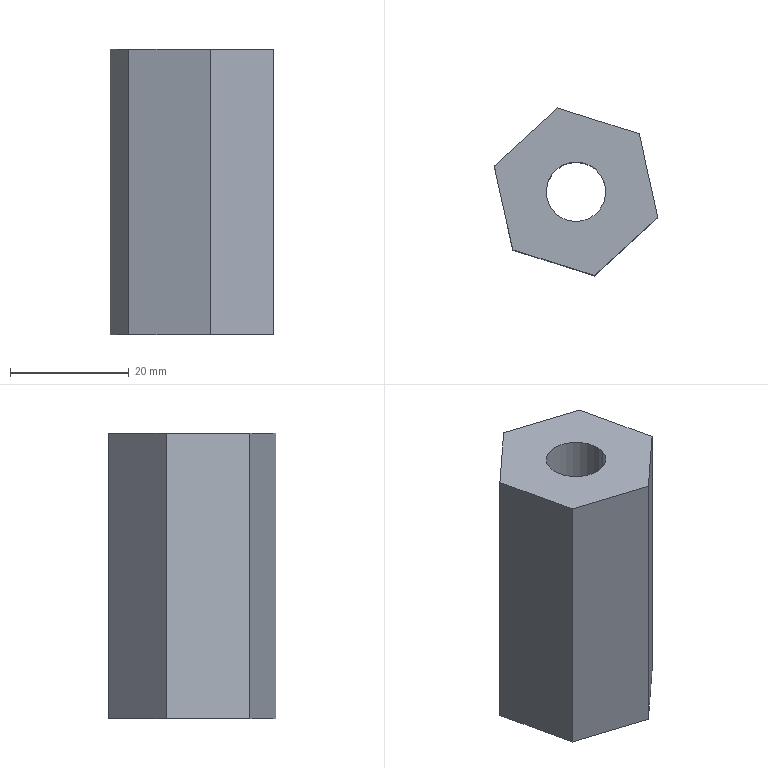Component | SolidWorks | ScraperSupport-1 | 1 solid | 10 faces | box 27.53 x 28.18 x 48 mm | volume 22211 mm3 | plane 8 | cylinder 2 | commonest cylinder face diameters 10 x2
STEP:
#1=COLOUR_RGB('',0.7922,0.8196,0.9333);
#2=FILL_AREA_STYLE_COLOUR('',#1);
#3=FILL_AREA_STYLE('',(#2));
#4=SURFACE_STYLE_FILL_AREA(#3);
#5=SURFACE_SIDE_STYLE('',(#4));
#6=SURFACE_STYLE_USAGE(.BOTH.,#5);
#7=PRESENTATION_STYLE_ASSIGNMENT((#6));
#8=CARTESIAN_POINT('',(20.038,-9.226,57.903));
#9=VERTEX_POINT('',#8);
#10=CARTESIAN_POINT('',(19.666,-9.098,57.903));
#11=VERTEX_POINT('',#10);
#12=CARTESIAN_POINT('',(19.852,-9.162,57.903));
#13=DIRECTION('',(-0.,-0.,-1.));
#14=DIRECTION('',(-0.9451,0.3269,0.));
#15=AXIS2_PLACEMENT_3D('',#12,#13,#14);
#16=CIRCLE('',#15,0.1969);
#17=EDGE_CURVE('',#9,#11,#16,.T.);
#18=ORIENTED_EDGE('',*,*,#17,.T.);
#19=CARTESIAN_POINT('',(19.666,-9.098,59.792));
#20=VERTEX_POINT('',#19);
#21=CARTESIAN_POINT('',(19.666,-9.098,57.903));
#22=DIRECTION('',(0.,0.,1.));
#23=VECTOR('',#22,39.37);
#24=LINE('',#21,#23);
#25=EDGE_CURVE('',#11,#20,#24,.T.);
#26=ORIENTED_EDGE('',*,*,#25,.T.);
#27=CARTESIAN_POINT('',(20.038,-9.226,59.792));
#28=VERTEX_POINT('',#27);
#29=CARTESIAN_POINT('',(19.852,-9.162,59.792));
#30=DIRECTION('',(-0.,-0.,-1.));
#31=DIRECTION('',(-0.9451,0.3269,0.));
#32=AXIS2_PLACEMENT_3D('',#29,#30,#31);
#33=CIRCLE('',#32,0.1969);
#34=EDGE_CURVE('',#28,#20,#33,.T.);
#35=ORIENTED_EDGE('',*,*,#34,.F.);
#36=CARTESIAN_POINT('',(20.038,-9.226,57.903));
#37=DIRECTION('',(0.,0.,1.));
#38=VECTOR('',#37,39.37);
#39=LINE('',#36,#38);
#40=EDGE_CURVE('',#9,#28,#39,.T.);
#41=ORIENTED_EDGE('',*,*,#40,.F.);
#42=EDGE_LOOP('',(#18,#26,#35,#41));
#43=FACE_OUTER_BOUND('',#42,.T.);
#44=CARTESIAN_POINT('',(19.852,-9.162,57.903));
#45=DIRECTION('',(0.,0.,1.));
#46=DIRECTION('',(0.9451,-0.3269,0.));
#47=AXIS2_PLACEMENT_3D('',#44,#45,#46);
#48=CYLINDRICAL_SURFACE('',#47,0.1969);
#49=ADVANCED_FACE('',(#43),#48,.F.);
#50=CARTESIAN_POINT('',(19.31,-8.991,57.903));
#51=VERTEX_POINT('',#50);
#52=CARTESIAN_POINT('',(19.729,-8.607,57.903));
#53=VERTEX_POINT('',#52);
#54=CARTESIAN_POINT('',(19.31,-8.991,57.903));
#55=DIRECTION('',(0.7374,0.6754,-0.));
#56=VECTOR('',#55,39.37);
#57=LINE('',#54,#56);
#58=EDGE_CURVE('',#51,#53,#57,.T.);
#59=ORIENTED_EDGE('',*,*,#58,.T.);
#60=CARTESIAN_POINT('',(20.271,-8.778,57.903));
#61=VERTEX_POINT('',#60);
#62=CARTESIAN_POINT('',(19.729,-8.607,57.903));
#63=DIRECTION('',(0.9537,-0.3009,-0.));
#64=VECTOR('',#63,39.37);
#65=LINE('',#62,#64);
#66=EDGE_CURVE('',#53,#61,#65,.T.);
#67=ORIENTED_EDGE('',*,*,#66,.T.);
#68=CARTESIAN_POINT('',(20.394,-9.333,57.903));
#69=VERTEX_POINT('',#68);
#70=CARTESIAN_POINT('',(20.271,-8.778,57.903));
#71=DIRECTION('',(0.2162,-0.9763,0.));
#72=VECTOR('',#71,39.37);
#73=LINE('',#70,#72);
#74=EDGE_CURVE('',#61,#69,#73,.T.);
#75=ORIENTED_EDGE('',*,*,#74,.T.);
#76=CARTESIAN_POINT('',(19.975,-9.717,57.903));
#77=VERTEX_POINT('',#76);
#78=CARTESIAN_POINT('',(20.394,-9.333,57.903));
#79=DIRECTION('',(-0.7374,-0.6754,0.));
#80=VECTOR('',#79,39.37);
#81=LINE('',#78,#80);
#82=EDGE_CURVE('',#69,#77,#81,.T.);
#83=ORIENTED_EDGE('',*,*,#82,.T.);
#84=CARTESIAN_POINT('',(19.433,-9.546,57.903));
#85=VERTEX_POINT('',#84);
#86=CARTESIAN_POINT('',(19.975,-9.717,57.903));
#87=DIRECTION('',(-0.9537,0.3009,0.));
#88=VECTOR('',#87,39.37);
#89=LINE('',#86,#88);
#90=EDGE_CURVE('',#77,#85,#89,.T.);
#91=ORIENTED_EDGE('',*,*,#90,.T.);
#92=CARTESIAN_POINT('',(19.433,-9.546,57.903));
#93=DIRECTION('',(-0.2162,0.9763,-0.));
#94=VECTOR('',#93,39.37);
#95=LINE('',#92,#94);
#96=EDGE_CURVE('',#85,#51,#95,.T.);
#97=ORIENTED_EDGE('',*,*,#96,.T.);
#98=EDGE_LOOP('',(#59,#67,#75,#83,#91,#97));
#99=FACE_OUTER_BOUND('',#98,.T.);
#100=ORIENTED_EDGE('',*,*,#17,.F.);
#101=CARTESIAN_POINT('',(19.852,-9.162,57.903));
#102=DIRECTION('',(-0.,-0.,-1.));
#103=DIRECTION('',(-0.9451,0.3269,0.));
#104=AXIS2_PLACEMENT_3D('',#101,#102,#103);
#105=CIRCLE('',#104,0.1969);
#106=EDGE_CURVE('',#11,#9,#105,.T.);
#107=ORIENTED_EDGE('',*,*,#106,.F.);
#108=EDGE_LOOP('',(#100,#107));
#109=FACE_BOUND('',#108,.T.);
#110=CARTESIAN_POINT('',(19.852,-9.162,57.903));
#111=DIRECTION('',(-0.,-0.,-1.));
#112=DIRECTION('',(-0.9451,0.3269,0.));
#113=AXIS2_PLACEMENT_3D('',#110,#111,#112);
#114=PLANE('',#113);
#115=ADVANCED_FACE('',(#99,#109),#114,.T.);
#116=CARTESIAN_POINT('',(19.31,-8.991,59.792));
#117=VERTEX_POINT('',#116);
#118=CARTESIAN_POINT('',(19.729,-8.607,59.792));
#119=VERTEX_POINT('',#118);
#120=CARTESIAN_POINT('',(19.31,-8.991,59.792));
#121=DIRECTION('',(0.7374,0.6754,-0.));
#122=VECTOR('',#121,39.37);
#123=LINE('',#120,#122);
#124=EDGE_CURVE('',#117,#119,#123,.T.);
#125=ORIENTED_EDGE('',*,*,#124,.F.);
#126=CARTESIAN_POINT('',(19.433,-9.546,59.792));
#127=VERTEX_POINT('',#126);
#128=CARTESIAN_POINT('',(19.433,-9.546,59.792));
#129=DIRECTION('',(-0.2162,0.9763,-0.));
#130=VECTOR('',#129,39.37);
#131=LINE('',#128,#130);
#132=EDGE_CURVE('',#127,#117,#131,.T.);
#133=ORIENTED_EDGE('',*,*,#132,.F.);
#134=CARTESIAN_POINT('',(19.975,-9.717,59.792));
#135=VERTEX_POINT('',#134);
#136=CARTESIAN_POINT('',(19.975,-9.717,59.792));
#137=DIRECTION('',(-0.9537,0.3009,0.));
#138=VECTOR('',#137,39.37);
#139=LINE('',#136,#138);
#140=EDGE_CURVE('',#135,#127,#139,.T.);
#141=ORIENTED_EDGE('',*,*,#140,.F.);
#142=CARTESIAN_POINT('',(20.394,-9.333,59.792));
#143=VERTEX_POINT('',#142);
#144=CARTESIAN_POINT('',(20.394,-9.333,59.792));
#145=DIRECTION('',(-0.7374,-0.6754,0.));
#146=VECTOR('',#145,39.37);
#147=LINE('',#144,#146);
#148=EDGE_CURVE('',#143,#135,#147,.T.);
#149=ORIENTED_EDGE('',*,*,#148,.F.);
#150=CARTESIAN_POINT('',(20.271,-8.778,59.792));
#151=VERTEX_POINT('',#150);
#152=CARTESIAN_POINT('',(20.271,-8.778,59.792));
#153=DIRECTION('',(0.2162,-0.9763,0.));
#154=VECTOR('',#153,39.37);
#155=LINE('',#152,#154);
#156=EDGE_CURVE('',#151,#143,#155,.T.);
#157=ORIENTED_EDGE('',*,*,#156,.F.);
#158=CARTESIAN_POINT('',(19.729,-8.607,59.792));
#159=DIRECTION('',(0.9537,-0.3009,-0.));
#160=VECTOR('',#159,39.37);
#161=LINE('',#158,#160);
#162=EDGE_CURVE('',#119,#151,#161,.T.);
#163=ORIENTED_EDGE('',*,*,#162,.F.);
#164=EDGE_LOOP('',(#125,#133,#141,#149,#157,#163));
#165=FACE_OUTER_BOUND('',#164,.T.);
#166=ORIENTED_EDGE('',*,*,#34,.T.);
#167=CARTESIAN_POINT('',(19.852,-9.162,59.792));
#168=DIRECTION('',(-0.,-0.,-1.));
#169=DIRECTION('',(-0.9451,0.3269,0.));
#170=AXIS2_PLACEMENT_3D('',#167,#168,#169);
#171=CIRCLE('',#170,0.1969);
#172=EDGE_CURVE('',#20,#28,#171,.T.);
#173=ORIENTED_EDGE('',*,*,#172,.T.);
#174=EDGE_LOOP('',(#166,#173));
#175=FACE_BOUND('',#174,.T.);
#176=CARTESIAN_POINT('',(19.852,-9.162,59.792));
#177=DIRECTION('',(-0.,-0.,-1.));
#178=DIRECTION('',(-0.9451,0.3269,0.));
#179=AXIS2_PLACEMENT_3D('',#176,#177,#178);
#180=PLANE('',#179);
#181=ADVANCED_FACE('',(#165,#175),#180,.F.);
#182=ORIENTED_EDGE('',*,*,#124,.T.);
#183=CARTESIAN_POINT('',(19.729,-8.607,57.903));
#184=DIRECTION('',(0.,0.,1.));
#185=VECTOR('',#184,39.37);
#186=LINE('',#183,#185);
#187=EDGE_CURVE('',#53,#119,#186,.T.);
#188=ORIENTED_EDGE('',*,*,#187,.F.);
#189=ORIENTED_EDGE('',*,*,#58,.F.);
#190=CARTESIAN_POINT('',(19.31,-8.991,57.903));
#191=DIRECTION('',(0.,0.,1.));
#192=VECTOR('',#191,39.37);
#193=LINE('',#190,#192);
#194=EDGE_CURVE('',#51,#117,#193,.T.);
#195=ORIENTED_EDGE('',*,*,#194,.T.);
#196=EDGE_LOOP('',(#182,#188,#189,#195));
#197=FACE_OUTER_BOUND('',#196,.T.);
#198=CARTESIAN_POINT('',(19.31,-8.991,57.903));
#199=DIRECTION('',(0.6754,-0.7374,0.));
#200=DIRECTION('',(-0.7374,-0.6754,0.));
#201=AXIS2_PLACEMENT_3D('',#198,#199,#200);
#202=PLANE('',#201);
#203=ADVANCED_FACE('',(#197),#202,.F.);
#204=ORIENTED_EDGE('',*,*,#162,.T.);
#205=CARTESIAN_POINT('',(20.271,-8.778,57.903));
#206=DIRECTION('',(0.,0.,1.));
#207=VECTOR('',#206,39.37);
#208=LINE('',#205,#207);
#209=EDGE_CURVE('',#61,#151,#208,.T.);
#210=ORIENTED_EDGE('',*,*,#209,.F.);
#211=ORIENTED_EDGE('',*,*,#66,.F.);
#212=ORIENTED_EDGE('',*,*,#187,.T.);
#213=EDGE_LOOP('',(#204,#210,#211,#212));
#214=FACE_OUTER_BOUND('',#213,.T.);
#215=CARTESIAN_POINT('',(19.729,-8.607,57.903));
#216=DIRECTION('',(-0.3009,-0.9537,0.));
#217=DIRECTION('',(-0.9537,0.3009,0.));
#218=AXIS2_PLACEMENT_3D('',#215,#216,#217);
#219=PLANE('',#218);
#220=ADVANCED_FACE('',(#214),#219,.F.);
#221=ORIENTED_EDGE('',*,*,#156,.T.);
#222=CARTESIAN_POINT('',(20.394,-9.333,57.903));
#223=DIRECTION('',(0.,0.,1.));
#224=VECTOR('',#223,39.37);
#225=LINE('',#222,#224);
#226=EDGE_CURVE('',#69,#143,#225,.T.);
#227=ORIENTED_EDGE('',*,*,#226,.F.);
#228=ORIENTED_EDGE('',*,*,#74,.F.);
#229=ORIENTED_EDGE('',*,*,#209,.T.);
#230=EDGE_LOOP('',(#221,#227,#228,#229));
#231=FACE_OUTER_BOUND('',#230,.T.);
#232=CARTESIAN_POINT('',(20.271,-8.778,57.903));
#233=DIRECTION('',(-0.9763,-0.2162,0.));
#234=DIRECTION('',(-0.2162,0.9763,-0.));
#235=AXIS2_PLACEMENT_3D('',#232,#233,#234);
#236=PLANE('',#235);
#237=ADVANCED_FACE('',(#231),#236,.F.);
#238=ORIENTED_EDGE('',*,*,#148,.T.);
#239=CARTESIAN_POINT('',(19.975,-9.717,57.903));
#240=DIRECTION('',(0.,0.,1.));
#241=VECTOR('',#240,39.37);
#242=LINE('',#239,#241);
#243=EDGE_CURVE('',#77,#135,#242,.T.);
#244=ORIENTED_EDGE('',*,*,#243,.F.);
#245=ORIENTED_EDGE('',*,*,#82,.F.);
#246=ORIENTED_EDGE('',*,*,#226,.T.);
#247=EDGE_LOOP('',(#238,#244,#245,#246));
#248=FACE_OUTER_BOUND('',#247,.T.);
#249=CARTESIAN_POINT('',(20.394,-9.333,57.903));
#250=DIRECTION('',(-0.6754,0.7374,-0.));
#251=DIRECTION('',(0.7374,0.6754,-0.));
#252=AXIS2_PLACEMENT_3D('',#249,#250,#251);
#253=PLANE('',#252);
#254=ADVANCED_FACE('',(#248),#253,.F.);
#255=ORIENTED_EDGE('',*,*,#140,.T.);
#256=CARTESIAN_POINT('',(19.433,-9.546,57.903));
#257=DIRECTION('',(0.,0.,1.));
#258=VECTOR('',#257,39.37);
#259=LINE('',#256,#258);
#260=EDGE_CURVE('',#85,#127,#259,.T.);
#261=ORIENTED_EDGE('',*,*,#260,.F.);
#262=ORIENTED_EDGE('',*,*,#90,.F.);
#263=ORIENTED_EDGE('',*,*,#243,.T.);
#264=EDGE_LOOP('',(#255,#261,#262,#263));
#265=FACE_OUTER_BOUND('',#264,.T.);
#266=CARTESIAN_POINT('',(19.975,-9.717,57.903));
#267=DIRECTION('',(0.3009,0.9537,-0.));
#268=DIRECTION('',(0.9537,-0.3009,-0.));
#269=AXIS2_PLACEMENT_3D('',#266,#267,#268);
#270=PLANE('',#269);
#271=ADVANCED_FACE('',(#265),#270,.F.);
#272=ORIENTED_EDGE('',*,*,#132,.T.);
#273=ORIENTED_EDGE('',*,*,#194,.F.);
#274=ORIENTED_EDGE('',*,*,#96,.F.);
#275=ORIENTED_EDGE('',*,*,#260,.T.);
#276=EDGE_LOOP('',(#272,#273,#274,#275));
#277=FACE_OUTER_BOUND('',#276,.T.);
#278=CARTESIAN_POINT('',(19.433,-9.546,57.903));
#279=DIRECTION('',(0.9763,0.2162,-0.));
#280=DIRECTION('',(0.2162,-0.9763,0.));
#281=AXIS2_PLACEMENT_3D('',#278,#279,#280);
#282=PLANE('',#281);
#283=ADVANCED_FACE('',(#277),#282,.F.);
#284=ORIENTED_EDGE('',*,*,#25,.F.);
#285=ORIENTED_EDGE('',*,*,#106,.T.);
#286=ORIENTED_EDGE('',*,*,#40,.T.);
#287=ORIENTED_EDGE('',*,*,#172,.F.);
#288=EDGE_LOOP('',(#284,#285,#286,#287));
#289=FACE_OUTER_BOUND('',#288,.T.);
#290=CARTESIAN_POINT('',(19.852,-9.162,57.903));
#291=DIRECTION('',(0.,0.,1.));
#292=DIRECTION('',(0.9451,-0.3269,0.));
#293=AXIS2_PLACEMENT_3D('',#290,#291,#292);
#294=CYLINDRICAL_SURFACE('',#293,0.1969);
#295=ADVANCED_FACE('',(#289),#294,.F.);
#296=CLOSED_SHELL('',(#49,#115,#181,#203,#220,#237,#254,#271,#283,#295));
#297=MANIFOLD_SOLID_BREP('',#296);
#298=STYLED_ITEM('',(#7),#297);
#299=PRESENTATION_LAYER_ASSIGNMENT('','',(#298));
#300=(LENGTH_UNIT()NAMED_UNIT(*)SI_UNIT($,.METRE.));
#301=LENGTH_MEASURE_WITH_UNIT(LENGTH_MEASURE(0.0254),#300);
#302=DIMENSIONAL_EXPONENTS(1.,0.,0.,0.,0.,0.,0.);
#303=(CONVERSION_BASED_UNIT('',#301)LENGTH_UNIT()NAMED_UNIT(#302));
#304=UNCERTAINTY_MEASURE_WITH_UNIT(LENGTH_MEASURE(0.00001),#303,'','');
#305=(NAMED_UNIT(*)PLANE_ANGLE_UNIT()SI_UNIT($,.RADIAN.));
#306=(NAMED_UNIT(*)SI_UNIT($,.STERADIAN.)SOLID_ANGLE_UNIT());
#307=(GEOMETRIC_REPRESENTATION_CONTEXT(3)GLOBAL_UNCERTAINTY_ASSIGNED_CONTEXT((#304))GLOBAL_UNIT_ASSIGNED_CONTEXT((#303,#305,#306))REPRESENTATION_CONTEXT('',''));
#308=MECHANICAL_DESIGN_GEOMETRIC_PRESENTATION_REPRESENTATION('',(#298),#307);
#309=CARTESIAN_POINT('',(0.,0.,0.));
#310=DIRECTION('',(0.,0.,1.));
#311=DIRECTION('',(1.,0.,0.));
#312=AXIS2_PLACEMENT_3D('',#309,#310,#311);
#313=(LENGTH_UNIT()NAMED_UNIT(*)SI_UNIT($,.METRE.));
#314=LENGTH_MEASURE_WITH_UNIT(LENGTH_MEASURE(0.0254),#313);
#315=DIMENSIONAL_EXPONENTS(1.,0.,0.,0.,0.,0.,0.);
#316=(CONVERSION_BASED_UNIT('',#314)LENGTH_UNIT()NAMED_UNIT(#315));
#317=UNCERTAINTY_MEASURE_WITH_UNIT(LENGTH_MEASURE(0.00001),#316,'','');
#318=(NAMED_UNIT(*)PLANE_ANGLE_UNIT()SI_UNIT($,.RADIAN.));
#319=(NAMED_UNIT(*)SI_UNIT($,.STERADIAN.)SOLID_ANGLE_UNIT());
#320=(GEOMETRIC_REPRESENTATION_CONTEXT(3)GLOBAL_UNCERTAINTY_ASSIGNED_CONTEXT((#317))GLOBAL_UNIT_ASSIGNED_CONTEXT((#316,#318,#319))REPRESENTATION_CONTEXT('',''));
#321=ADVANCED_BREP_SHAPE_REPRESENTATION('',(#297,#312),#320);